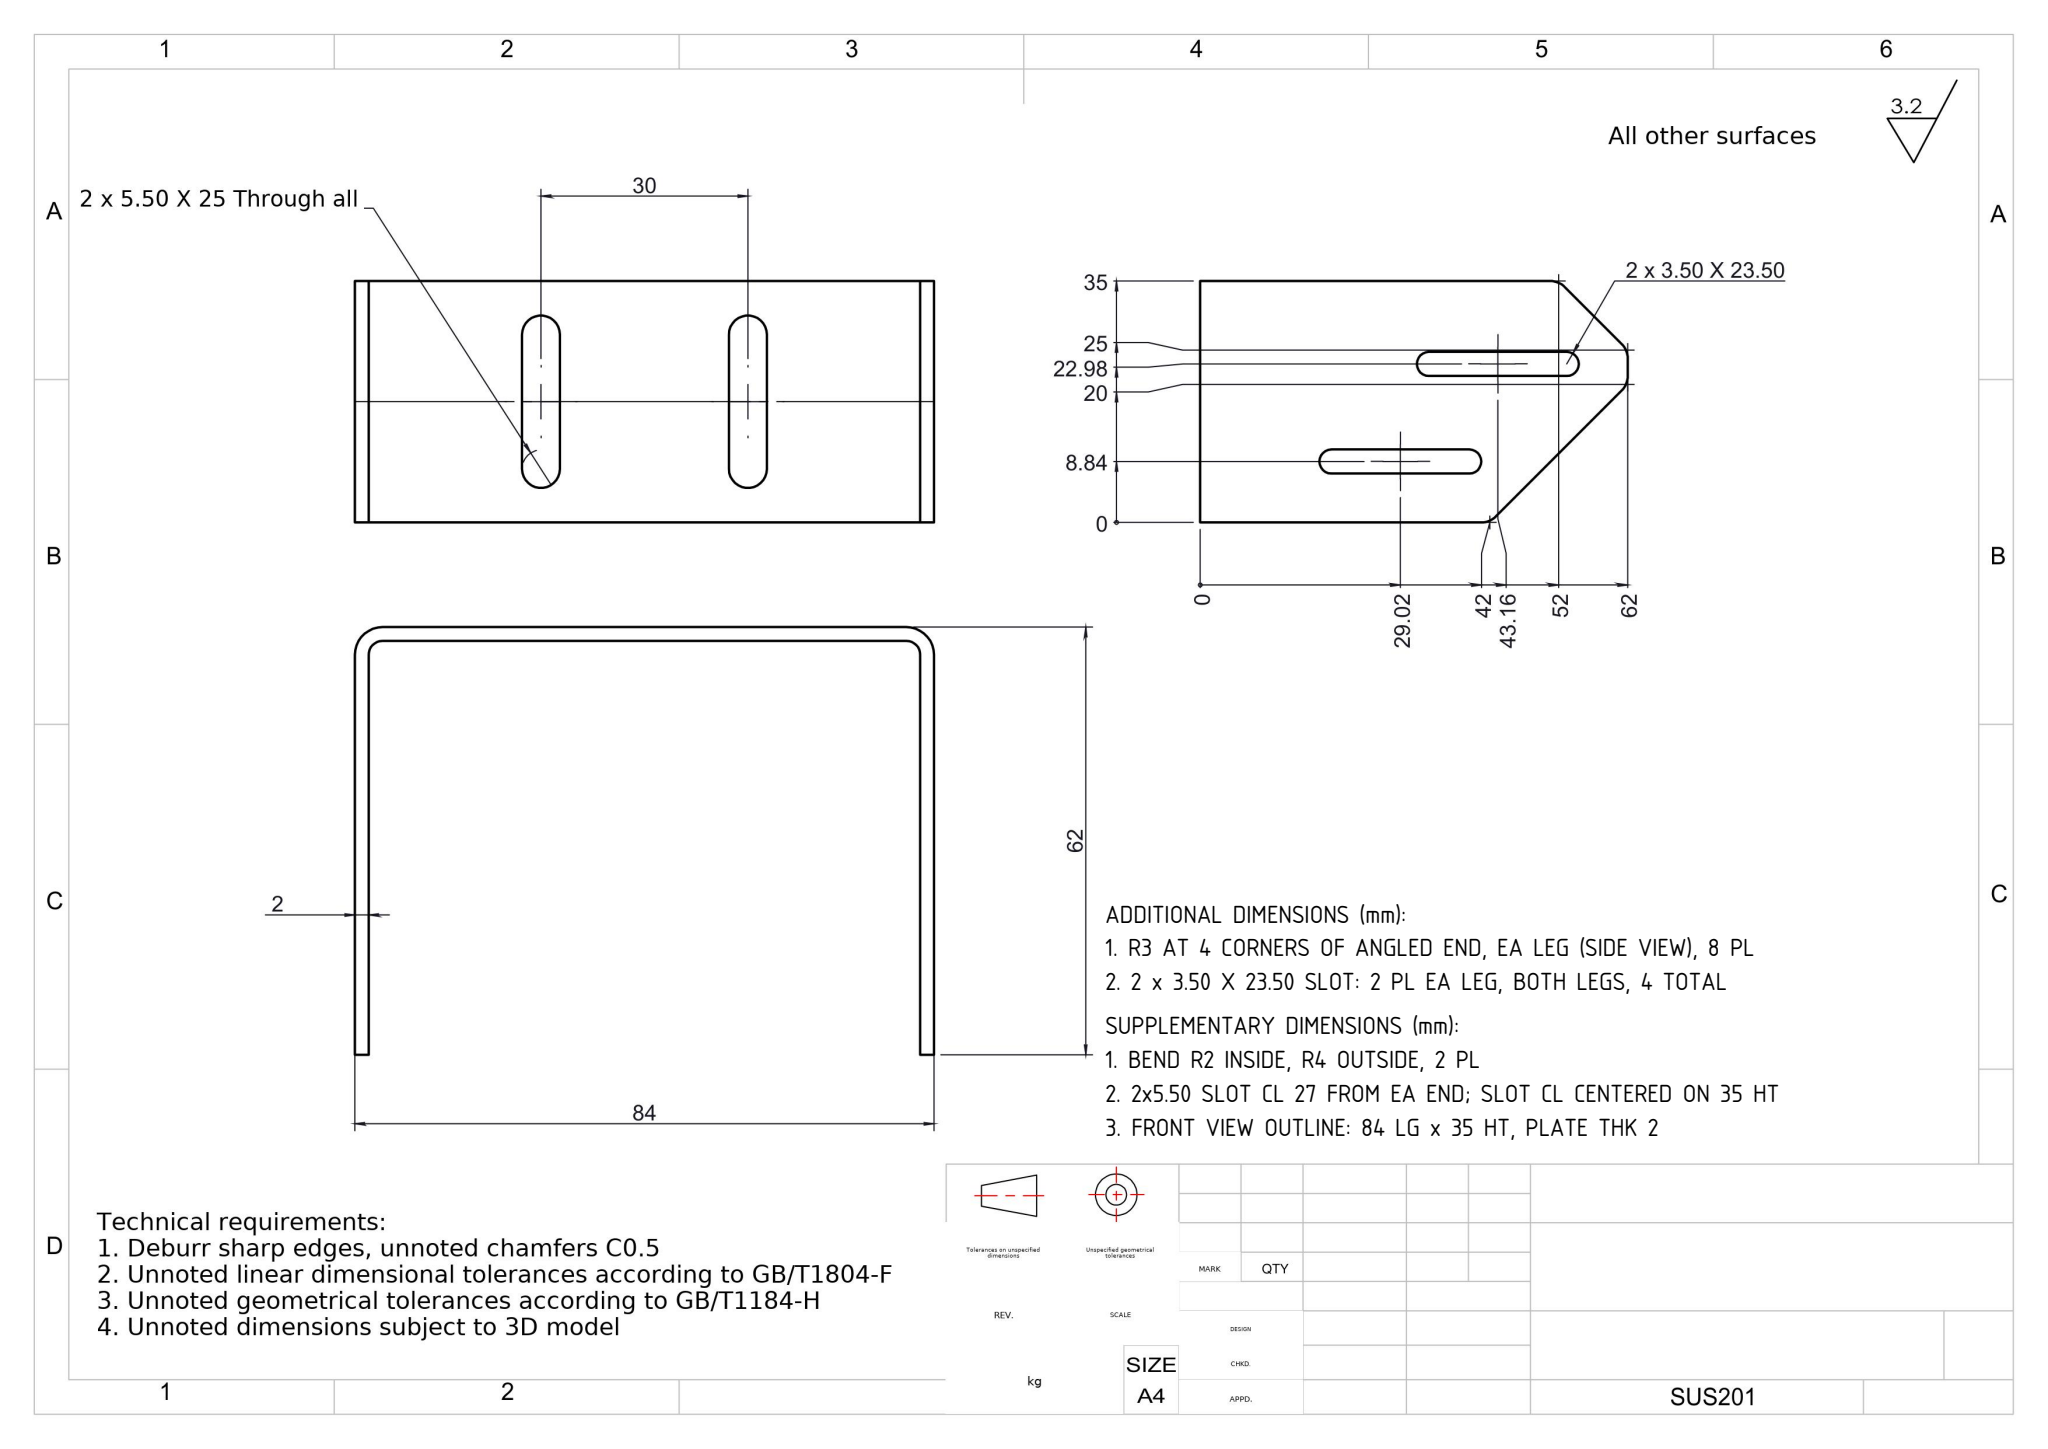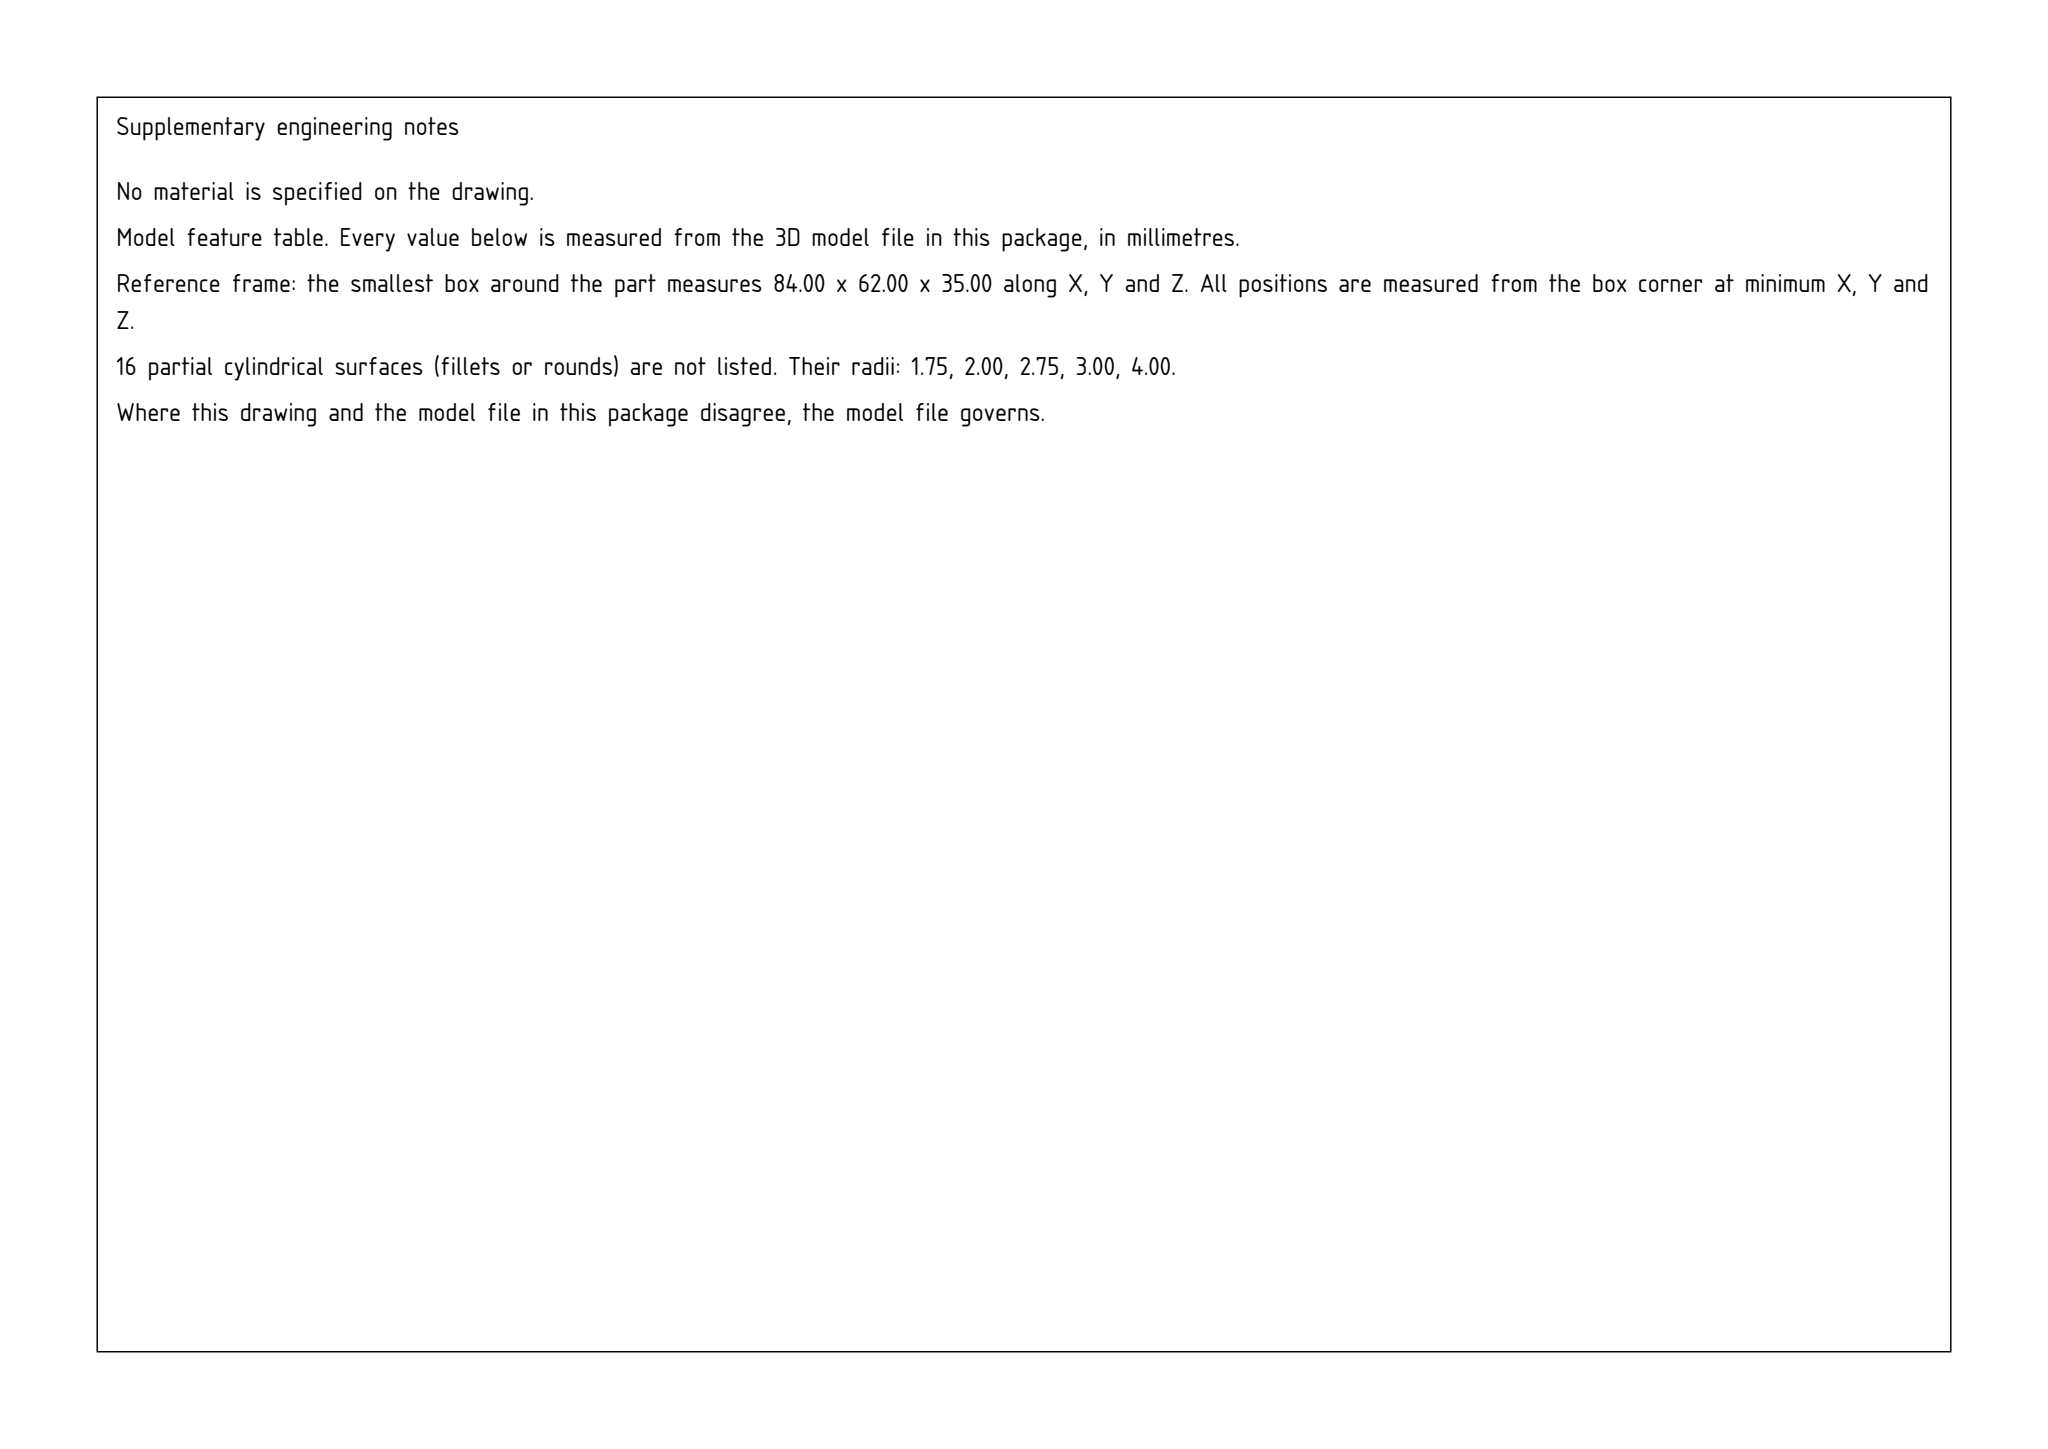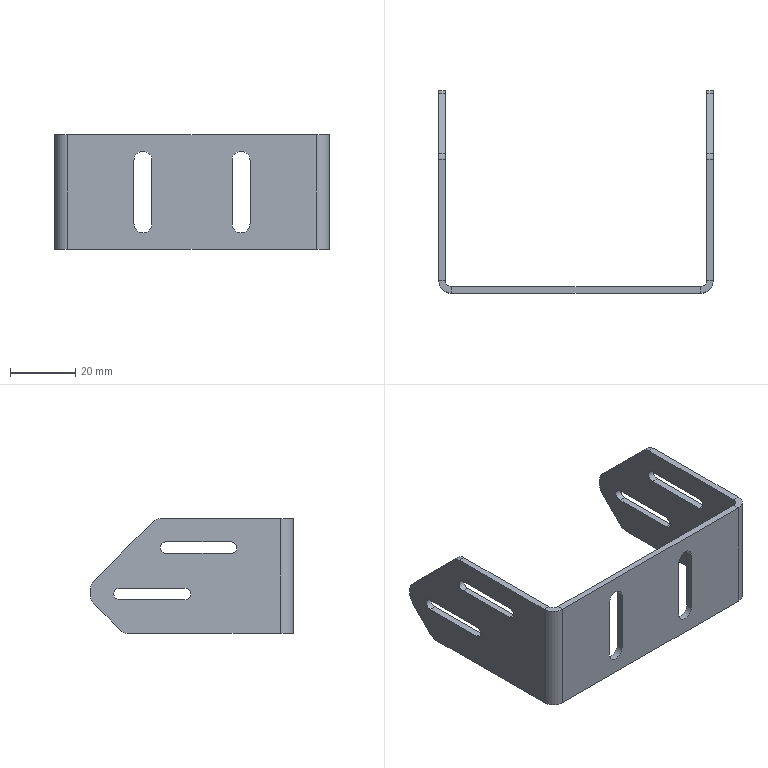Part | SolidWorks | mm | 1 solid | 64 faces | box 84 x 62 x 35 mm | volume 11936 mm3 | plane 34 | cylinder 30 | commonest cylinder face diameters 3.5 x12 6 x8 5.5 x6 4 x2 8 x2